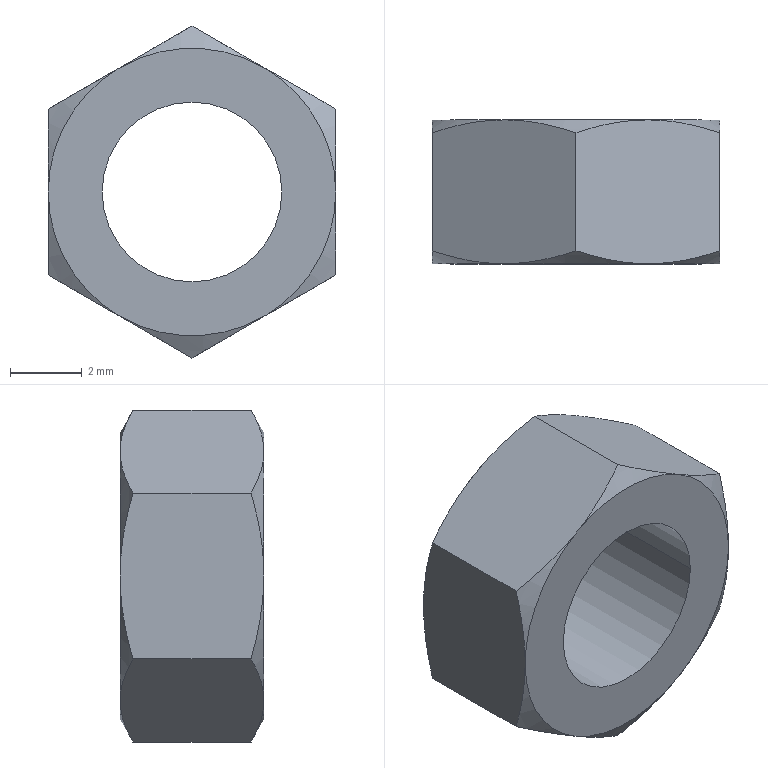Component | SolidWorks | PB_16x75_S_U_FA_M_2_0-1_164nut1-1 | 1 solid | 22 faces | box 8 x 4 x 9.24 mm | volume 142 mm3 | cone 12 | plane 8 | cylinder 2 | commonest cylinder face diameters 5 x2
build123d program:
from build123d import *

# Parameters (mm, degrees)
EXTRUDE1_DEPTH          = 2
EXTRUDE1_DEPTH_BACK     = 2
SKETCH3_W               = 16
SKETCH3_H               = 16
CUT_EXTRUDE1_DEPTH      = 7.429
CUT_EXTRUDE1_DEPTH_BACK = 7.429
SKETCH4_R               = 2.5


with BuildPart() as part:
    # Sketch1 → Revolve1 (revolve)
    with BuildSketch(Plane.XY, mode=Mode.PRIVATE) as revolve1_sk:
        Polygon((-2, 0), (-2, 4), (-1.538, 4.8), (1.538, 4.8), (2, 4), (2, 0), align=None)
    revolve(revolve1_sk.sketch.rotate(Axis((2, 0, 0), (-1, 0, 0)), 270), axis=Axis((2, 0, 0), (-1, 0, 0)))

    # Sketch2 → Cut-Revolve1 (revolve, cut)
    with BuildSketch(Plane.XY, mode=Mode.PRIVATE) as cut_revolve1_sk:
        Polygon((-2, 0), (-2, 2.5), (-1.567, 2.067), (1.567, 2.067), (2, 2.5), (2, 0), align=None)
    revolve(cut_revolve1_sk.sketch.rotate(Axis((2, 0, 0), (-1, 0, 0)), 270), axis=Axis((2, 0, 0), (-1, 0, 0)), mode=Mode.SUBTRACT)

    # Sketch3 → Extrude1 (cut, two sides: drawn at the far end of the back side and taken through both)
    with BuildSketch(Plane(origin=(0, 0, 0), x_dir=(0, 0, -1), z_dir=(1, 0, 0)).offset(-EXTRUDE1_DEPTH_BACK)):
        Rectangle(SKETCH3_W, SKETCH3_H)
        Polygon((-4, 2.309), (-4, -2.309), (0, -4.619), (4, -2.309), (4, 2.309), (0, 4.619), align=None, mode=Mode.SUBTRACT)
    extrude(amount=EXTRUDE1_DEPTH + EXTRUDE1_DEPTH_BACK, mode=Mode.SUBTRACT)

    # Sketch4 → Cut-Extrude1 (cut, two sides: drawn at the far end of the back side and taken through both)
    with BuildSketch(Plane(origin=(0, 0, 0), x_dir=(0, 0, -1), z_dir=(1, 0, 0)).offset(-CUT_EXTRUDE1_DEPTH_BACK)):
        Circle(SKETCH4_R)
    extrude(amount=CUT_EXTRUDE1_DEPTH + CUT_EXTRUDE1_DEPTH_BACK, mode=Mode.SUBTRACT)


solid = part.part

# Placed as in the assembly
solid = solid.moved(Location((45, -241, 55), (90, -90, 0)))
STEP:
#1=COLOUR_RGB('',0.7922,0.8196,0.9333);
#2=FILL_AREA_STYLE_COLOUR('',#1);
#3=FILL_AREA_STYLE('',(#2));
#4=SURFACE_STYLE_FILL_AREA(#3);
#5=SURFACE_SIDE_STYLE('',(#4));
#6=SURFACE_STYLE_USAGE(.BOTH.,#5);
#7=PRESENTATION_STYLE_ASSIGNMENT((#6));
#8=CARTESIAN_POINT('',(1.673,-9.567,2.165));
#9=VERTEX_POINT('',#8);
#10=CARTESIAN_POINT('',(1.87,-9.567,2.165));
#11=VERTEX_POINT('',#10);
#12=CARTESIAN_POINT('',(1.772,-9.567,2.165));
#13=DIRECTION('',(0.,1.,0.));
#14=DIRECTION('',(1.,0.,0.));
#15=AXIS2_PLACEMENT_3D('',#12,#13,#14);
#16=CIRCLE('',#15,0.09843);
#17=EDGE_CURVE('',#9,#11,#16,.T.);
#18=ORIENTED_EDGE('',*,*,#17,.F.);
#19=CARTESIAN_POINT('',(1.673,-9.409,2.165));
#20=VERTEX_POINT('',#19);
#21=CARTESIAN_POINT('',(1.673,-9.567,2.165));
#22=DIRECTION('',(0.,1.,0.));
#23=VECTOR('',#22,39.37);
#24=LINE('',#21,#23);
#25=EDGE_CURVE('',#9,#20,#24,.T.);
#26=ORIENTED_EDGE('',*,*,#25,.T.);
#27=CARTESIAN_POINT('',(1.87,-9.409,2.165));
#28=VERTEX_POINT('',#27);
#29=CARTESIAN_POINT('',(1.772,-9.409,2.165));
#30=DIRECTION('',(0.,1.,0.));
#31=DIRECTION('',(1.,0.,0.));
#32=AXIS2_PLACEMENT_3D('',#29,#30,#31);
#33=CIRCLE('',#32,0.09843);
#34=EDGE_CURVE('',#20,#28,#33,.T.);
#35=ORIENTED_EDGE('',*,*,#34,.T.);
#36=CARTESIAN_POINT('',(1.87,-9.567,2.165));
#37=DIRECTION('',(0.,1.,0.));
#38=VECTOR('',#37,39.37);
#39=LINE('',#36,#38);
#40=EDGE_CURVE('',#11,#28,#39,.T.);
#41=ORIENTED_EDGE('',*,*,#40,.F.);
#42=EDGE_LOOP('',(#18,#26,#35,#41));
#43=FACE_OUTER_BOUND('',#42,.T.);
#44=CARTESIAN_POINT('',(1.772,-9.567,2.165));
#45=DIRECTION('',(0.,1.,0.));
#46=DIRECTION('',(1.,0.,0.));
#47=AXIS2_PLACEMENT_3D('',#44,#45,#46);
#48=CYLINDRICAL_SURFACE('',#47,0.09843);
#49=ADVANCED_FACE('',(#43),#48,.F.);
#50=CARTESIAN_POINT('',(1.929,-9.553,2.256));
#51=VERTEX_POINT('',#50);
#52=CARTESIAN_POINT('',(1.929,-9.567,2.165));
#53=VERTEX_POINT('',#52);
#54=CARTESIAN_POINT('',(1.929,-9.553,2.256));
#55=CARTESIAN_POINT('',(1.929,-9.557,2.241));
#56=CARTESIAN_POINT('',(1.929,-9.561,2.226));
#57=CARTESIAN_POINT('',(1.929,-9.566,2.196));
#58=CARTESIAN_POINT('',(1.929,-9.567,2.181));
#59=CARTESIAN_POINT('',(1.929,-9.567,2.165));
#60=B_SPLINE_CURVE_WITH_KNOTS('',3,(#54,#55,#56,#57,#58,#59),.UNSPECIFIED.,.F.,.F.,(4,2,4),(0.004136,0.005305,0.006473),.UNSPECIFIED.);
#61=EDGE_CURVE('',#51,#53,#60,.T.);
#62=ORIENTED_EDGE('',*,*,#61,.F.);
#63=CARTESIAN_POINT('',(1.85,-9.567,2.302));
#64=VERTEX_POINT('',#63);
#65=CARTESIAN_POINT('',(1.85,-9.567,2.302));
#66=CARTESIAN_POINT('',(1.864,-9.567,2.294));
#67=CARTESIAN_POINT('',(1.877,-9.566,2.286));
#68=CARTESIAN_POINT('',(1.903,-9.561,2.271));
#69=CARTESIAN_POINT('',(1.916,-9.557,2.264));
#70=CARTESIAN_POINT('',(1.929,-9.553,2.256));
#71=B_SPLINE_CURVE_WITH_KNOTS('',3,(#65,#66,#67,#68,#69,#70),.UNSPECIFIED.,.F.,.F.,(4,2,4),(0.002337,0.003501,0.004665),.UNSPECIFIED.);
#72=EDGE_CURVE('',#64,#51,#71,.T.);
#73=ORIENTED_EDGE('',*,*,#72,.F.);
#74=CARTESIAN_POINT('',(1.772,-9.567,2.165));
#75=DIRECTION('',(0.,-1.,0.));
#76=DIRECTION('',(-1.,0.,0.));
#77=AXIS2_PLACEMENT_3D('',#74,#75,#76);
#78=CIRCLE('',#77,0.1575);
#79=EDGE_CURVE('',#53,#64,#78,.T.);
#80=ORIENTED_EDGE('',*,*,#79,.F.);
#81=EDGE_LOOP('',(#62,#73,#80));
#82=FACE_OUTER_BOUND('',#81,.T.);
#83=CARTESIAN_POINT('',(1.772,-9.549,2.165));
#84=DIRECTION('',(0.,1.,0.));
#85=DIRECTION('',(1.,0.,0.));
#86=AXIS2_PLACEMENT_3D('',#83,#84,#85);
#87=CONICAL_SURFACE('',#86,0.189,1.047);
#88=ADVANCED_FACE('',(#82),#87,.T.);
#89=CARTESIAN_POINT('',(1.929,-9.553,2.074));
#90=VERTEX_POINT('',#89);
#91=CARTESIAN_POINT('',(1.929,-9.567,2.165));
#92=CARTESIAN_POINT('',(1.929,-9.567,2.15));
#93=CARTESIAN_POINT('',(1.929,-9.566,2.134));
#94=CARTESIAN_POINT('',(1.929,-9.561,2.104));
#95=CARTESIAN_POINT('',(1.929,-9.557,2.089));
#96=CARTESIAN_POINT('',(1.929,-9.553,2.074));
#97=B_SPLINE_CURVE_WITH_KNOTS('',3,(#91,#92,#93,#94,#95,#96),.UNSPECIFIED.,.F.,.F.,(4,2,4),(0.006473,0.007642,0.008811),.UNSPECIFIED.);
#98=EDGE_CURVE('',#53,#90,#97,.T.);
#99=ORIENTED_EDGE('',*,*,#98,.F.);
#100=CARTESIAN_POINT('',(1.85,-9.567,2.029));
#101=VERTEX_POINT('',#100);
#102=CARTESIAN_POINT('',(1.772,-9.567,2.165));
#103=DIRECTION('',(0.,-1.,0.));
#104=DIRECTION('',(-1.,0.,0.));
#105=AXIS2_PLACEMENT_3D('',#102,#103,#104);
#106=CIRCLE('',#105,0.1575);
#107=EDGE_CURVE('',#101,#53,#106,.T.);
#108=ORIENTED_EDGE('',*,*,#107,.F.);
#109=CARTESIAN_POINT('',(1.929,-9.553,2.074));
#110=CARTESIAN_POINT('',(1.903,-9.561,2.06));
#111=CARTESIAN_POINT('',(1.877,-9.567,2.044));
#112=CARTESIAN_POINT('',(1.85,-9.567,2.029));
#113=B_SPLINE_CURVE_WITH_KNOTS('',3,(#109,#110,#111,#112),.UNSPECIFIED.,.F.,.F.,(4,4),(0.00000024,0.002337),.UNSPECIFIED.);
#114=EDGE_CURVE('',#90,#101,#113,.T.);
#115=ORIENTED_EDGE('',*,*,#114,.F.);
#116=EDGE_LOOP('',(#99,#108,#115));
#117=FACE_OUTER_BOUND('',#116,.T.);
#118=CARTESIAN_POINT('',(1.772,-9.549,2.165));
#119=DIRECTION('',(0.,1.,0.));
#120=DIRECTION('',(1.,0.,0.));
#121=AXIS2_PLACEMENT_3D('',#118,#119,#120);
#122=CONICAL_SURFACE('',#121,0.189,1.047);
#123=ADVANCED_FACE('',(#117),#122,.T.);
#124=CARTESIAN_POINT('',(1.772,-9.553,1.984));
#125=VERTEX_POINT('',#124);
#126=CARTESIAN_POINT('',(1.85,-9.567,2.029));
#127=CARTESIAN_POINT('',(1.837,-9.567,2.021));
#128=CARTESIAN_POINT('',(1.824,-9.566,2.014));
#129=CARTESIAN_POINT('',(1.797,-9.561,1.998));
#130=CARTESIAN_POINT('',(1.785,-9.557,1.991));
#131=CARTESIAN_POINT('',(1.772,-9.553,1.984));
#132=B_SPLINE_CURVE_WITH_KNOTS('',3,(#126,#127,#128,#129,#130,#131),.UNSPECIFIED.,.F.,.F.,(4,2,4),(0.002337,0.003501,0.004665),.UNSPECIFIED.);
#133=EDGE_CURVE('',#101,#125,#132,.T.);
#134=ORIENTED_EDGE('',*,*,#133,.F.);
#135=CARTESIAN_POINT('',(1.693,-9.567,2.029));
#136=VERTEX_POINT('',#135);
#137=CARTESIAN_POINT('',(1.772,-9.567,2.165));
#138=DIRECTION('',(0.,-1.,0.));
#139=DIRECTION('',(-1.,0.,0.));
#140=AXIS2_PLACEMENT_3D('',#137,#138,#139);
#141=CIRCLE('',#140,0.1575);
#142=EDGE_CURVE('',#136,#101,#141,.T.);
#143=ORIENTED_EDGE('',*,*,#142,.F.);
#144=CARTESIAN_POINT('',(1.772,-9.553,1.984));
#145=CARTESIAN_POINT('',(1.746,-9.561,1.998));
#146=CARTESIAN_POINT('',(1.72,-9.567,2.013));
#147=CARTESIAN_POINT('',(1.693,-9.567,2.029));
#148=B_SPLINE_CURVE_WITH_KNOTS('',3,(#144,#145,#146,#147),.UNSPECIFIED.,.F.,.F.,(4,4),(0.00000024,0.002337),.UNSPECIFIED.);
#149=EDGE_CURVE('',#125,#136,#148,.T.);
#150=ORIENTED_EDGE('',*,*,#149,.F.);
#151=EDGE_LOOP('',(#134,#143,#150));
#152=FACE_OUTER_BOUND('',#151,.T.);
#153=CARTESIAN_POINT('',(1.772,-9.549,2.165));
#154=DIRECTION('',(0.,1.,0.));
#155=DIRECTION('',(1.,0.,0.));
#156=AXIS2_PLACEMENT_3D('',#153,#154,#155);
#157=CONICAL_SURFACE('',#156,0.189,1.047);
#158=ADVANCED_FACE('',(#152),#157,.T.);
#159=CARTESIAN_POINT('',(1.772,-9.553,2.347));
#160=VERTEX_POINT('',#159);
#161=CARTESIAN_POINT('',(1.772,-9.553,2.347));
#162=CARTESIAN_POINT('',(1.797,-9.561,2.332));
#163=CARTESIAN_POINT('',(1.824,-9.567,2.317));
#164=CARTESIAN_POINT('',(1.85,-9.567,2.302));
#165=B_SPLINE_CURVE_WITH_KNOTS('',3,(#161,#162,#163,#164),.UNSPECIFIED.,.F.,.F.,(4,4),(0.00000024,0.002337),.UNSPECIFIED.);
#166=EDGE_CURVE('',#160,#64,#165,.T.);
#167=ORIENTED_EDGE('',*,*,#166,.F.);
#168=CARTESIAN_POINT('',(1.693,-9.567,2.302));
#169=VERTEX_POINT('',#168);
#170=CARTESIAN_POINT('',(1.693,-9.567,2.302));
#171=CARTESIAN_POINT('',(1.706,-9.567,2.309));
#172=CARTESIAN_POINT('',(1.72,-9.566,2.317));
#173=CARTESIAN_POINT('',(1.746,-9.561,2.332));
#174=CARTESIAN_POINT('',(1.759,-9.557,2.34));
#175=CARTESIAN_POINT('',(1.772,-9.553,2.347));
#176=B_SPLINE_CURVE_WITH_KNOTS('',3,(#170,#171,#172,#173,#174,#175),.UNSPECIFIED.,.F.,.F.,(4,2,4),(0.002337,0.003501,0.004665),.UNSPECIFIED.);
#177=EDGE_CURVE('',#169,#160,#176,.T.);
#178=ORIENTED_EDGE('',*,*,#177,.F.);
#179=CARTESIAN_POINT('',(1.772,-9.567,2.165));
#180=DIRECTION('',(0.,-1.,0.));
#181=DIRECTION('',(-1.,0.,0.));
#182=AXIS2_PLACEMENT_3D('',#179,#180,#181);
#183=CIRCLE('',#182,0.1575);
#184=EDGE_CURVE('',#64,#169,#183,.T.);
#185=ORIENTED_EDGE('',*,*,#184,.F.);
#186=EDGE_LOOP('',(#167,#178,#185));
#187=FACE_OUTER_BOUND('',#186,.T.);
#188=CARTESIAN_POINT('',(1.772,-9.549,2.165));
#189=DIRECTION('',(0.,1.,0.));
#190=DIRECTION('',(1.,0.,0.));
#191=AXIS2_PLACEMENT_3D('',#188,#189,#190);
#192=CONICAL_SURFACE('',#191,0.189,1.047);
#193=ADVANCED_FACE('',(#187),#192,.T.);
#194=CARTESIAN_POINT('',(1.614,-9.553,2.074));
#195=VERTEX_POINT('',#194);
#196=CARTESIAN_POINT('',(1.693,-9.567,2.029));
#197=CARTESIAN_POINT('',(1.68,-9.567,2.037));
#198=CARTESIAN_POINT('',(1.666,-9.566,2.044));
#199=CARTESIAN_POINT('',(1.64,-9.561,2.06));
#200=CARTESIAN_POINT('',(1.627,-9.557,2.067));
#201=CARTESIAN_POINT('',(1.614,-9.553,2.074));
#202=B_SPLINE_CURVE_WITH_KNOTS('',3,(#196,#197,#198,#199,#200,#201),.UNSPECIFIED.,.F.,.F.,(4,2,4),(0.002337,0.003501,0.004665),.UNSPECIFIED.);
#203=EDGE_CURVE('',#136,#195,#202,.T.);
#204=ORIENTED_EDGE('',*,*,#203,.F.);
#205=CARTESIAN_POINT('',(1.614,-9.567,2.165));
#206=VERTEX_POINT('',#205);
#207=CARTESIAN_POINT('',(1.772,-9.567,2.165));
#208=DIRECTION('',(0.,-1.,0.));
#209=DIRECTION('',(-1.,0.,0.));
#210=AXIS2_PLACEMENT_3D('',#207,#208,#209);
#211=CIRCLE('',#210,0.1575);
#212=EDGE_CURVE('',#206,#136,#211,.T.);
#213=ORIENTED_EDGE('',*,*,#212,.F.);
#214=CARTESIAN_POINT('',(1.614,-9.553,2.074));
#215=CARTESIAN_POINT('',(1.614,-9.557,2.089));
#216=CARTESIAN_POINT('',(1.614,-9.561,2.104));
#217=CARTESIAN_POINT('',(1.614,-9.566,2.134));
#218=CARTESIAN_POINT('',(1.614,-9.567,2.15));
#219=CARTESIAN_POINT('',(1.614,-9.567,2.165));
#220=B_SPLINE_CURVE_WITH_KNOTS('',3,(#214,#215,#216,#217,#218,#219),.UNSPECIFIED.,.F.,.F.,(4,2,4),(0.01014,0.01131,0.01248),.UNSPECIFIED.);
#221=EDGE_CURVE('',#195,#206,#220,.T.);
#222=ORIENTED_EDGE('',*,*,#221,.F.);
#223=EDGE_LOOP('',(#204,#213,#222));
#224=FACE_OUTER_BOUND('',#223,.T.);
#225=CARTESIAN_POINT('',(1.772,-9.549,2.165));
#226=DIRECTION('',(0.,1.,0.));
#227=DIRECTION('',(1.,0.,0.));
#228=AXIS2_PLACEMENT_3D('',#225,#226,#227);
#229=CONICAL_SURFACE('',#228,0.189,1.047);
#230=ADVANCED_FACE('',(#224),#229,.T.);
#231=CARTESIAN_POINT('',(1.614,-9.553,2.256));
#232=VERTEX_POINT('',#231);
#233=CARTESIAN_POINT('',(1.614,-9.553,2.256));
#234=CARTESIAN_POINT('',(1.64,-9.561,2.271));
#235=CARTESIAN_POINT('',(1.666,-9.567,2.286));
#236=CARTESIAN_POINT('',(1.693,-9.567,2.302));
#237=B_SPLINE_CURVE_WITH_KNOTS('',3,(#233,#234,#235,#236),.UNSPECIFIED.,.F.,.F.,(4,4),(0.00000024,0.002337),.UNSPECIFIED.);
#238=EDGE_CURVE('',#232,#169,#237,.T.);
#239=ORIENTED_EDGE('',*,*,#238,.F.);
#240=CARTESIAN_POINT('',(1.614,-9.567,2.165));
#241=CARTESIAN_POINT('',(1.614,-9.567,2.181));
#242=CARTESIAN_POINT('',(1.614,-9.566,2.196));
#243=CARTESIAN_POINT('',(1.614,-9.561,2.226));
#244=CARTESIAN_POINT('',(1.614,-9.557,2.241));
#245=CARTESIAN_POINT('',(1.614,-9.553,2.256));
#246=B_SPLINE_CURVE_WITH_KNOTS('',3,(#240,#241,#242,#243,#244,#245),.UNSPECIFIED.,.F.,.F.,(4,2,4),(0.01248,0.01365,0.01482),.UNSPECIFIED.);
#247=EDGE_CURVE('',#206,#232,#246,.T.);
#248=ORIENTED_EDGE('',*,*,#247,.F.);
#249=CARTESIAN_POINT('',(1.772,-9.567,2.165));
#250=DIRECTION('',(0.,-1.,0.));
#251=DIRECTION('',(-1.,0.,0.));
#252=AXIS2_PLACEMENT_3D('',#249,#250,#251);
#253=CIRCLE('',#252,0.1575);
#254=EDGE_CURVE('',#169,#206,#253,.T.);
#255=ORIENTED_EDGE('',*,*,#254,.F.);
#256=EDGE_LOOP('',(#239,#248,#255));
#257=FACE_OUTER_BOUND('',#256,.T.);
#258=CARTESIAN_POINT('',(1.772,-9.549,2.165));
#259=DIRECTION('',(0.,1.,0.));
#260=DIRECTION('',(1.,0.,0.));
#261=AXIS2_PLACEMENT_3D('',#258,#259,#260);
#262=CONICAL_SURFACE('',#261,0.189,1.047);
#263=ADVANCED_FACE('',(#257),#262,.T.);
#264=CARTESIAN_POINT('',(1.614,-9.424,2.074));
#265=VERTEX_POINT('',#264);
#266=CARTESIAN_POINT('',(1.693,-9.409,2.029));
#267=VERTEX_POINT('',#266);
#268=CARTESIAN_POINT('',(1.614,-9.424,2.074));
#269=CARTESIAN_POINT('',(1.64,-9.415,2.06));
#270=CARTESIAN_POINT('',(1.666,-9.409,2.044));
#271=CARTESIAN_POINT('',(1.693,-9.409,2.029));
#272=B_SPLINE_CURVE_WITH_KNOTS('',3,(#268,#269,#270,#271),.UNSPECIFIED.,.F.,.F.,(4,4),(0.00000024,0.002337),.UNSPECIFIED.);
#273=EDGE_CURVE('',#265,#267,#272,.T.);
#274=ORIENTED_EDGE('',*,*,#273,.F.);
#275=CARTESIAN_POINT('',(1.614,-9.409,2.165));
#276=VERTEX_POINT('',#275);
#277=CARTESIAN_POINT('',(1.614,-9.409,2.165));
#278=CARTESIAN_POINT('',(1.614,-9.409,2.15));
#279=CARTESIAN_POINT('',(1.614,-9.411,2.134));
#280=CARTESIAN_POINT('',(1.614,-9.416,2.104));
#281=CARTESIAN_POINT('',(1.614,-9.419,2.089));
#282=CARTESIAN_POINT('',(1.614,-9.424,2.074));
#283=B_SPLINE_CURVE_WITH_KNOTS('',3,(#277,#278,#279,#280,#281,#282),.UNSPECIFIED.,.F.,.F.,(4,2,4),(0.006473,0.007642,0.008811),.UNSPECIFIED.);
#284=EDGE_CURVE('',#276,#265,#283,.T.);
#285=ORIENTED_EDGE('',*,*,#284,.F.);
#286=CARTESIAN_POINT('',(1.772,-9.409,2.165));
#287=DIRECTION('',(0.,-1.,0.));
#288=DIRECTION('',(-1.,0.,0.));
#289=AXIS2_PLACEMENT_3D('',#286,#287,#288);
#290=CIRCLE('',#289,0.1575);
#291=EDGE_CURVE('',#276,#267,#290,.T.);
#292=ORIENTED_EDGE('',*,*,#291,.T.);
#293=EDGE_LOOP('',(#274,#285,#292));
#294=FACE_OUTER_BOUND('',#293,.T.);
#295=CARTESIAN_POINT('',(1.772,-9.409,2.165));
#296=DIRECTION('',(0.,-1.,0.));
#297=DIRECTION('',(-1.,0.,0.));
#298=AXIS2_PLACEMENT_3D('',#295,#296,#297);
#299=CONICAL_SURFACE('',#298,0.1575,1.047);
#300=ADVANCED_FACE('',(#294),#299,.T.);
#301=CARTESIAN_POINT('',(1.772,-9.424,1.984));
#302=VERTEX_POINT('',#301);
#303=CARTESIAN_POINT('',(1.693,-9.409,2.029));
#304=CARTESIAN_POINT('',(1.706,-9.409,2.021));
#305=CARTESIAN_POINT('',(1.72,-9.411,2.014));
#306=CARTESIAN_POINT('',(1.746,-9.416,1.998));
#307=CARTESIAN_POINT('',(1.759,-9.419,1.991));
#308=CARTESIAN_POINT('',(1.772,-9.424,1.984));
#309=B_SPLINE_CURVE_WITH_KNOTS('',3,(#303,#304,#305,#306,#307,#308),.UNSPECIFIED.,.F.,.F.,(4,2,4),(0.002337,0.003501,0.004665),.UNSPECIFIED.);
#310=EDGE_CURVE('',#267,#302,#309,.T.);
#311=ORIENTED_EDGE('',*,*,#310,.F.);
#312=CARTESIAN_POINT('',(1.85,-9.409,2.029));
#313=VERTEX_POINT('',#312);
#314=CARTESIAN_POINT('',(1.772,-9.409,2.165));
#315=DIRECTION('',(0.,-1.,0.));
#316=DIRECTION('',(-1.,0.,0.));
#317=AXIS2_PLACEMENT_3D('',#314,#315,#316);
#318=CIRCLE('',#317,0.1575);
#319=EDGE_CURVE('',#267,#313,#318,.T.);
#320=ORIENTED_EDGE('',*,*,#319,.T.);
#321=CARTESIAN_POINT('',(1.772,-9.424,1.984));
#322=CARTESIAN_POINT('',(1.797,-9.415,1.998));
#323=CARTESIAN_POINT('',(1.824,-9.409,2.013));
#324=CARTESIAN_POINT('',(1.85,-9.409,2.029));
#325=B_SPLINE_CURVE_WITH_KNOTS('',3,(#321,#322,#323,#324),.UNSPECIFIED.,.F.,.F.,(4,4),(0.00000024,0.002337),.UNSPECIFIED.);
#326=EDGE_CURVE('',#302,#313,#325,.T.);
#327=ORIENTED_EDGE('',*,*,#326,.F.);
#328=EDGE_LOOP('',(#311,#320,#327));
#329=FACE_OUTER_BOUND('',#328,.T.);
#330=CARTESIAN_POINT('',(1.772,-9.409,2.165));
#331=DIRECTION('',(0.,-1.,0.));
#332=DIRECTION('',(-1.,0.,0.));
#333=AXIS2_PLACEMENT_3D('',#330,#331,#332);
#334=CONICAL_SURFACE('',#333,0.1575,1.047);
#335=ADVANCED_FACE('',(#329),#334,.T.);
#336=CARTESIAN_POINT('',(1.929,-9.424,2.074));
#337=VERTEX_POINT('',#336);
#338=CARTESIAN_POINT('',(1.85,-9.409,2.029));
#339=CARTESIAN_POINT('',(1.864,-9.409,2.037));
#340=CARTESIAN_POINT('',(1.877,-9.411,2.044));
#341=CARTESIAN_POINT('',(1.903,-9.416,2.06));
#342=CARTESIAN_POINT('',(1.916,-9.419,2.067));
#343=CARTESIAN_POINT('',(1.929,-9.424,2.074));
#344=B_SPLINE_CURVE_WITH_KNOTS('',3,(#338,#339,#340,#341,#342,#343),.UNSPECIFIED.,.F.,.F.,(4,2,4),(0.002337,0.003501,0.004665),.UNSPECIFIED.);
#345=EDGE_CURVE('',#313,#337,#344,.T.);
#346=ORIENTED_EDGE('',*,*,#345,.F.);
#347=CARTESIAN_POINT('',(1.929,-9.409,2.165));
#348=VERTEX_POINT('',#347);
#349=CARTESIAN_POINT('',(1.772,-9.409,2.165));
#350=DIRECTION('',(0.,-1.,0.));
#351=DIRECTION('',(-1.,0.,0.));
#352=AXIS2_PLACEMENT_3D('',#349,#350,#351);
#353=CIRCLE('',#352,0.1575);
#354=EDGE_CURVE('',#313,#348,#353,.T.);
#355=ORIENTED_EDGE('',*,*,#354,.T.);
#356=CARTESIAN_POINT('',(1.929,-9.424,2.074));
#357=CARTESIAN_POINT('',(1.929,-9.419,2.089));
#358=CARTESIAN_POINT('',(1.929,-9.416,2.104));
#359=CARTESIAN_POINT('',(1.929,-9.411,2.134));
#360=CARTESIAN_POINT('',(1.929,-9.409,2.15));
#361=CARTESIAN_POINT('',(1.929,-9.409,2.165));
#362=B_SPLINE_CURVE_WITH_KNOTS('',3,(#356,#357,#358,#359,#360,#361),.UNSPECIFIED.,.F.,.F.,(4,2,4),(0.01014,0.01131,0.01248),.UNSPECIFIED.);
#363=EDGE_CURVE('',#337,#348,#362,.T.);
#364=ORIENTED_EDGE('',*,*,#363,.F.);
#365=EDGE_LOOP('',(#346,#355,#364));
#366=FACE_OUTER_BOUND('',#365,.T.);
#367=CARTESIAN_POINT('',(1.772,-9.409,2.165));
#368=DIRECTION('',(0.,-1.,0.));
#369=DIRECTION('',(-1.,0.,0.));
#370=AXIS2_PLACEMENT_3D('',#367,#368,#369);
#371=CONICAL_SURFACE('',#370,0.1575,1.047);
#372=ADVANCED_FACE('',(#366),#371,.T.);
#373=CARTESIAN_POINT('',(1.929,-9.424,2.256));
#374=VERTEX_POINT('',#373);
#375=CARTESIAN_POINT('',(1.929,-9.409,2.165));
#376=CARTESIAN_POINT('',(1.929,-9.409,2.181));
#377=CARTESIAN_POINT('',(1.929,-9.411,2.196));
#378=CARTESIAN_POINT('',(1.929,-9.416,2.226));
#379=CARTESIAN_POINT('',(1.929,-9.419,2.241));
#380=CARTESIAN_POINT('',(1.929,-9.424,2.256));
#381=B_SPLINE_CURVE_WITH_KNOTS('',3,(#375,#376,#377,#378,#379,#380),.UNSPECIFIED.,.F.,.F.,(4,2,4),(0.01248,0.01365,0.01482),.UNSPECIFIED.);
#382=EDGE_CURVE('',#348,#374,#381,.T.);
#383=ORIENTED_EDGE('',*,*,#382,.F.);
#384=CARTESIAN_POINT('',(1.85,-9.409,2.302));
#385=VERTEX_POINT('',#384);
#386=CARTESIAN_POINT('',(1.772,-9.409,2.165));
#387=DIRECTION('',(0.,-1.,0.));
#388=DIRECTION('',(-1.,0.,0.));
#389=AXIS2_PLACEMENT_3D('',#386,#387,#388);
#390=CIRCLE('',#389,0.1575);
#391=EDGE_CURVE('',#348,#385,#390,.T.);
#392=ORIENTED_EDGE('',*,*,#391,.T.);
#393=CARTESIAN_POINT('',(1.929,-9.424,2.256));
#394=CARTESIAN_POINT('',(1.903,-9.415,2.271));
#395=CARTESIAN_POINT('',(1.877,-9.409,2.286));
#396=CARTESIAN_POINT('',(1.85,-9.409,2.302));
#397=B_SPLINE_CURVE_WITH_KNOTS('',3,(#393,#394,#395,#396),.UNSPECIFIED.,.F.,.F.,(4,4),(0.00000024,0.002337),.UNSPECIFIED.);
#398=EDGE_CURVE('',#374,#385,#397,.T.);
#399=ORIENTED_EDGE('',*,*,#398,.F.);
#400=EDGE_LOOP('',(#383,#392,#399));
#401=FACE_OUTER_BOUND('',#400,.T.);
#402=CARTESIAN_POINT('',(1.772,-9.409,2.165));
#403=DIRECTION('',(0.,-1.,0.));
#404=DIRECTION('',(-1.,0.,0.));
#405=AXIS2_PLACEMENT_3D('',#402,#403,#404);
#406=CONICAL_SURFACE('',#405,0.1575,1.047);
#407=ADVANCED_FACE('',(#401),#406,.T.);
#408=CARTESIAN_POINT('',(1.772,-9.424,2.347));
#409=VERTEX_POINT('',#408);
#410=CARTESIAN_POINT('',(1.85,-9.409,2.302));
#411=CARTESIAN_POINT('',(1.837,-9.409,2.309));
#412=CARTESIAN_POINT('',(1.824,-9.411,2.317));
#413=CARTESIAN_POINT('',(1.797,-9.416,2.332));
#414=CARTESIAN_POINT('',(1.785,-9.419,2.34));
#415=CARTESIAN_POINT('',(1.772,-9.424,2.347));
#416=B_SPLINE_CURVE_WITH_KNOTS('',3,(#410,#411,#412,#413,#414,#415),.UNSPECIFIED.,.F.,.F.,(4,2,4),(0.002337,0.003501,0.004665),.UNSPECIFIED.);
#417=EDGE_CURVE('',#385,#409,#416,.T.);
#418=ORIENTED_EDGE('',*,*,#417,.F.);
#419=CARTESIAN_POINT('',(1.693,-9.409,2.302));
#420=VERTEX_POINT('',#419);
#421=CARTESIAN_POINT('',(1.772,-9.409,2.165));
#422=DIRECTION('',(0.,-1.,0.));
#423=DIRECTION('',(-1.,0.,0.));
#424=AXIS2_PLACEMENT_3D('',#421,#422,#423);
#425=CIRCLE('',#424,0.1575);
#426=EDGE_CURVE('',#385,#420,#425,.T.);
#427=ORIENTED_EDGE('',*,*,#426,.T.);
#428=CARTESIAN_POINT('',(1.772,-9.424,2.347));
#429=CARTESIAN_POINT('',(1.746,-9.415,2.332));
#430=CARTESIAN_POINT('',(1.72,-9.409,2.317));
#431=CARTESIAN_POINT('',(1.693,-9.409,2.302));
#432=B_SPLINE_CURVE_WITH_KNOTS('',3,(#428,#429,#430,#431),.UNSPECIFIED.,.F.,.F.,(4,4),(0.00000024,0.002337),.UNSPECIFIED.);
#433=EDGE_CURVE('',#409,#420,#432,.T.);
#434=ORIENTED_EDGE('',*,*,#433,.F.);
#435=EDGE_LOOP('',(#418,#427,#434));
#436=FACE_OUTER_BOUND('',#435,.T.);
#437=CARTESIAN_POINT('',(1.772,-9.409,2.165));
#438=DIRECTION('',(0.,-1.,0.));
#439=DIRECTION('',(-1.,0.,0.));
#440=AXIS2_PLACEMENT_3D('',#437,#438,#439);
#441=CONICAL_SURFACE('',#440,0.1575,1.047);
#442=ADVANCED_FACE('',(#436),#441,.T.);
#443=CARTESIAN_POINT('',(1.614,-9.424,2.256));
#444=VERTEX_POINT('',#443);
#445=CARTESIAN_POINT('',(1.693,-9.409,2.302));
#446=CARTESIAN_POINT('',(1.68,-9.409,2.294));
#447=CARTESIAN_POINT('',(1.666,-9.411,2.286));
#448=CARTESIAN_POINT('',(1.64,-9.416,2.271));
#449=CARTESIAN_POINT('',(1.627,-9.419,2.264));
#450=CARTESIAN_POINT('',(1.614,-9.424,2.256));
#451=B_SPLINE_CURVE_WITH_KNOTS('',3,(#445,#446,#447,#448,#449,#450),.UNSPECIFIED.,.F.,.F.,(4,2,4),(0.002337,0.003501,0.004665),.UNSPECIFIED.);
#452=EDGE_CURVE('',#420,#444,#451,.T.);
#453=ORIENTED_EDGE('',*,*,#452,.F.);
#454=CARTESIAN_POINT('',(1.772,-9.409,2.165));
#455=DIRECTION('',(0.,-1.,0.));
#456=DIRECTION('',(-1.,0.,0.));
#457=AXIS2_PLACEMENT_3D('',#454,#455,#456);
#458=CIRCLE('',#457,0.1575);
#459=EDGE_CURVE('',#420,#276,#458,.T.);
#460=ORIENTED_EDGE('',*,*,#459,.T.);
#461=CARTESIAN_POINT('',(1.614,-9.424,2.256));
#462=CARTESIAN_POINT('',(1.614,-9.419,2.241));
#463=CARTESIAN_POINT('',(1.614,-9.416,2.226));
#464=CARTESIAN_POINT('',(1.614,-9.411,2.196));
#465=CARTESIAN_POINT('',(1.614,-9.409,2.181));
#466=CARTESIAN_POINT('',(1.614,-9.409,2.165));
#467=B_SPLINE_CURVE_WITH_KNOTS('',3,(#461,#462,#463,#464,#465,#466),.UNSPECIFIED.,.F.,.F.,(4,2,4),(0.004136,0.005305,0.006473),.UNSPECIFIED.);
#468=EDGE_CURVE('',#444,#276,#467,.T.);
#469=ORIENTED_EDGE('',*,*,#468,.F.);
#470=EDGE_LOOP('',(#453,#460,#469));
#471=FACE_OUTER_BOUND('',#470,.T.);
#472=CARTESIAN_POINT('',(1.772,-9.409,2.165));
#473=DIRECTION('',(0.,-1.,0.));
#474=DIRECTION('',(-1.,0.,0.));
#475=AXIS2_PLACEMENT_3D('',#472,#473,#474);
#476=CONICAL_SURFACE('',#475,0.1575,1.047);
#477=ADVANCED_FACE('',(#471),#476,.T.);
#478=ORIENTED_EDGE('',*,*,#212,.T.);
#479=ORIENTED_EDGE('',*,*,#142,.T.);
#480=ORIENTED_EDGE('',*,*,#107,.T.);
#481=ORIENTED_EDGE('',*,*,#79,.T.);
#482=ORIENTED_EDGE('',*,*,#184,.T.);
#483=ORIENTED_EDGE('',*,*,#254,.T.);
#484=EDGE_LOOP('',(#478,#479,#480,#481,#482,#483));
#485=FACE_OUTER_BOUND('',#484,.T.);
#486=CARTESIAN_POINT('',(1.772,-9.567,2.165));
#487=DIRECTION('',(0.,1.,0.));
#488=DIRECTION('',(1.,0.,0.));
#489=AXIS2_PLACEMENT_3D('',#486,#487,#488);
#490=CIRCLE('',#489,0.09843);
#491=EDGE_CURVE('',#11,#9,#490,.T.);
#492=ORIENTED_EDGE('',*,*,#491,.T.);
#493=ORIENTED_EDGE('',*,*,#17,.T.);
#494=EDGE_LOOP('',(#492,#493));
#495=FACE_BOUND('',#494,.T.);
#496=CARTESIAN_POINT('',(1.772,-9.567,2.165));
#497=DIRECTION('',(0.,1.,0.));
#498=DIRECTION('',(1.,0.,0.));
#499=AXIS2_PLACEMENT_3D('',#496,#497,#498);
#500=PLANE('',#499);
#501=ADVANCED_FACE('',(#485,#495),#500,.F.);
#502=ORIENTED_EDGE('',*,*,#291,.F.);
#503=ORIENTED_EDGE('',*,*,#459,.F.);
#504=ORIENTED_EDGE('',*,*,#426,.F.);
#505=ORIENTED_EDGE('',*,*,#391,.F.);
#506=ORIENTED_EDGE('',*,*,#354,.F.);
#507=ORIENTED_EDGE('',*,*,#319,.F.);
#508=EDGE_LOOP('',(#502,#503,#504,#505,#506,#507));
#509=FACE_OUTER_BOUND('',#508,.T.);
#510=CARTESIAN_POINT('',(1.772,-9.409,2.165));
#511=DIRECTION('',(0.,1.,0.));
#512=DIRECTION('',(1.,0.,0.));
#513=AXIS2_PLACEMENT_3D('',#510,#511,#512);
#514=CIRCLE('',#513,0.09843);
#515=EDGE_CURVE('',#28,#20,#514,.T.);
#516=ORIENTED_EDGE('',*,*,#515,.F.);
#517=ORIENTED_EDGE('',*,*,#34,.F.);
#518=EDGE_LOOP('',(#516,#517));
#519=FACE_BOUND('',#518,.T.);
#520=CARTESIAN_POINT('',(1.772,-9.409,2.008));
#521=DIRECTION('',(0.,-1.,0.));
#522=DIRECTION('',(-1.,0.,0.));
#523=AXIS2_PLACEMENT_3D('',#520,#521,#522);
#524=PLANE('',#523);
#525=ADVANCED_FACE('',(#509,#519),#524,.F.);
#526=ORIENTED_EDGE('',*,*,#149,.T.);
#527=ORIENTED_EDGE('',*,*,#203,.T.);
#528=CARTESIAN_POINT('',(1.614,-9.567,2.074));
#529=DIRECTION('',(0.,1.,0.));
#530=VECTOR('',#529,39.37);
#531=LINE('',#528,#530);
#532=EDGE_CURVE('',#195,#265,#531,.T.);
#533=ORIENTED_EDGE('',*,*,#532,.T.);
#534=ORIENTED_EDGE('',*,*,#273,.T.);
#535=ORIENTED_EDGE('',*,*,#310,.T.);
#536=CARTESIAN_POINT('',(1.772,-9.567,1.984));
#537=DIRECTION('',(0.,1.,0.));
#538=VECTOR('',#537,39.37);
#539=LINE('',#536,#538);
#540=EDGE_CURVE('',#125,#302,#539,.T.);
#541=ORIENTED_EDGE('',*,*,#540,.F.);
#542=EDGE_LOOP('',(#526,#527,#533,#534,#535,#541));
#543=FACE_OUTER_BOUND('',#542,.T.);
#544=CARTESIAN_POINT('',(1.772,-9.567,1.984));
#545=DIRECTION('',(-0.5,0.,-0.866));
#546=DIRECTION('',(-0.866,0.,0.5));
#547=AXIS2_PLACEMENT_3D('',#544,#545,#546);
#548=PLANE('',#547);
#549=ADVANCED_FACE('',(#543),#548,.T.);
#550=ORIENTED_EDGE('',*,*,#114,.T.);
#551=ORIENTED_EDGE('',*,*,#133,.T.);
#552=ORIENTED_EDGE('',*,*,#540,.T.);
#553=ORIENTED_EDGE('',*,*,#326,.T.);
#554=ORIENTED_EDGE('',*,*,#345,.T.);
#555=CARTESIAN_POINT('',(1.929,-9.567,2.074));
#556=DIRECTION('',(0.,1.,0.));
#557=VECTOR('',#556,39.37);
#558=LINE('',#555,#557);
#559=EDGE_CURVE('',#90,#337,#558,.T.);
#560=ORIENTED_EDGE('',*,*,#559,.F.);
#561=EDGE_LOOP('',(#550,#551,#552,#553,#554,#560));
#562=FACE_OUTER_BOUND('',#561,.T.);
#563=CARTESIAN_POINT('',(1.929,-9.567,2.074));
#564=DIRECTION('',(0.5,0.,-0.866));
#565=DIRECTION('',(-0.866,0.,-0.5));
#566=AXIS2_PLACEMENT_3D('',#563,#564,#565);
#567=PLANE('',#566);
#568=ADVANCED_FACE('',(#562),#567,.T.);
#569=ORIENTED_EDGE('',*,*,#61,.T.);
#570=ORIENTED_EDGE('',*,*,#98,.T.);
#571=ORIENTED_EDGE('',*,*,#559,.T.);
#572=ORIENTED_EDGE('',*,*,#363,.T.);
#573=ORIENTED_EDGE('',*,*,#382,.T.);
#574=CARTESIAN_POINT('',(1.929,-9.567,2.256));
#575=DIRECTION('',(0.,1.,0.));
#576=VECTOR('',#575,39.37);
#577=LINE('',#574,#576);
#578=EDGE_CURVE('',#51,#374,#577,.T.);
#579=ORIENTED_EDGE('',*,*,#578,.F.);
#580=EDGE_LOOP('',(#569,#570,#571,#572,#573,#579));
#581=FACE_OUTER_BOUND('',#580,.T.);
#582=CARTESIAN_POINT('',(1.929,-9.567,2.256));
#583=DIRECTION('',(1.,0.,0.));
#584=DIRECTION('',(0.,-1.,0.));
#585=AXIS2_PLACEMENT_3D('',#582,#583,#584);
#586=PLANE('',#585);
#587=ADVANCED_FACE('',(#581),#586,.T.);
#588=ORIENTED_EDGE('',*,*,#166,.T.);
#589=ORIENTED_EDGE('',*,*,#72,.T.);
#590=ORIENTED_EDGE('',*,*,#578,.T.);
#591=ORIENTED_EDGE('',*,*,#398,.T.);
#592=ORIENTED_EDGE('',*,*,#417,.T.);
#593=CARTESIAN_POINT('',(1.772,-9.567,2.347));
#594=DIRECTION('',(0.,1.,0.));
#595=VECTOR('',#594,39.37);
#596=LINE('',#593,#595);
#597=EDGE_CURVE('',#160,#409,#596,.T.);
#598=ORIENTED_EDGE('',*,*,#597,.F.);
#599=EDGE_LOOP('',(#588,#589,#590,#591,#592,#598));
#600=FACE_OUTER_BOUND('',#599,.T.);
#601=CARTESIAN_POINT('',(1.772,-9.567,2.347));
#602=DIRECTION('',(0.5,0.,0.866));
#603=DIRECTION('',(0.866,0.,-0.5));
#604=AXIS2_PLACEMENT_3D('',#601,#602,#603);
#605=PLANE('',#604);
#606=ADVANCED_FACE('',(#600),#605,.T.);
#607=ORIENTED_EDGE('',*,*,#238,.T.);
#608=ORIENTED_EDGE('',*,*,#177,.T.);
#609=ORIENTED_EDGE('',*,*,#597,.T.);
#610=ORIENTED_EDGE('',*,*,#433,.T.);
#611=ORIENTED_EDGE('',*,*,#452,.T.);
#612=CARTESIAN_POINT('',(1.614,-9.567,2.256));
#613=DIRECTION('',(0.,1.,0.));
#614=VECTOR('',#613,39.37);
#615=LINE('',#612,#614);
#616=EDGE_CURVE('',#232,#444,#615,.T.);
#617=ORIENTED_EDGE('',*,*,#616,.F.);
#618=EDGE_LOOP('',(#607,#608,#609,#610,#611,#617));
#619=FACE_OUTER_BOUND('',#618,.T.);
#620=CARTESIAN_POINT('',(1.614,-9.567,2.256));
#621=DIRECTION('',(-0.5,0.,0.866));
#622=DIRECTION('',(0.866,0.,0.5));
#623=AXIS2_PLACEMENT_3D('',#620,#621,#622);
#624=PLANE('',#623);
#625=ADVANCED_FACE('',(#619),#624,.T.);
#626=ORIENTED_EDGE('',*,*,#221,.T.);
#627=ORIENTED_EDGE('',*,*,#247,.T.);
#628=ORIENTED_EDGE('',*,*,#616,.T.);
#629=ORIENTED_EDGE('',*,*,#468,.T.);
#630=ORIENTED_EDGE('',*,*,#284,.T.);
#631=ORIENTED_EDGE('',*,*,#532,.F.);
#632=EDGE_LOOP('',(#626,#627,#628,#629,#630,#631));
#633=FACE_OUTER_BOUND('',#632,.T.);
#634=CARTESIAN_POINT('',(1.614,-9.567,2.074));
#635=DIRECTION('',(-1.,0.,0.));
#636=DIRECTION('',(0.,1.,0.));
#637=AXIS2_PLACEMENT_3D('',#634,#635,#636);
#638=PLANE('',#637);
#639=ADVANCED_FACE('',(#633),#638,.T.);
#640=ORIENTED_EDGE('',*,*,#25,.F.);
#641=ORIENTED_EDGE('',*,*,#491,.F.);
#642=ORIENTED_EDGE('',*,*,#40,.T.);
#643=ORIENTED_EDGE('',*,*,#515,.T.);
#644=EDGE_LOOP('',(#640,#641,#642,#643));
#645=FACE_OUTER_BOUND('',#644,.T.);
#646=CARTESIAN_POINT('',(1.772,-9.567,2.165));
#647=DIRECTION('',(0.,1.,0.));
#648=DIRECTION('',(1.,0.,0.));
#649=AXIS2_PLACEMENT_3D('',#646,#647,#648);
#650=CYLINDRICAL_SURFACE('',#649,0.09843);
#651=ADVANCED_FACE('',(#645),#650,.F.);
#652=CLOSED_SHELL('',(#49,#88,#123,#158,#193,#230,#263,#300,#335,#372,#407,#442,#477,#501,#525,#549,#568,#587,#606,#625,#639,#651));
#653=MANIFOLD_SOLID_BREP('',#652);
#654=STYLED_ITEM('',(#7),#653);
#655=PRESENTATION_LAYER_ASSIGNMENT('','',(#654));
#656=(LENGTH_UNIT()NAMED_UNIT(*)SI_UNIT($,.METRE.));
#657=LENGTH_MEASURE_WITH_UNIT(LENGTH_MEASURE(0.0254),#656);
#658=DIMENSIONAL_EXPONENTS(1.,0.,0.,0.,0.,0.,0.);
#659=(CONVERSION_BASED_UNIT('',#657)LENGTH_UNIT()NAMED_UNIT(#658));
#660=UNCERTAINTY_MEASURE_WITH_UNIT(LENGTH_MEASURE(0.00001),#659,'','');
#661=(NAMED_UNIT(*)PLANE_ANGLE_UNIT()SI_UNIT($,.RADIAN.));
#662=(NAMED_UNIT(*)SI_UNIT($,.STERADIAN.)SOLID_ANGLE_UNIT());
#663=(GEOMETRIC_REPRESENTATION_CONTEXT(3)GLOBAL_UNCERTAINTY_ASSIGNED_CONTEXT((#660))GLOBAL_UNIT_ASSIGNED_CONTEXT((#659,#661,#662))REPRESENTATION_CONTEXT('',''));
#664=MECHANICAL_DESIGN_GEOMETRIC_PRESENTATION_REPRESENTATION('',(#654),#663);
#665=CARTESIAN_POINT('',(0.,0.,0.));
#666=DIRECTION('',(0.,0.,1.));
#667=DIRECTION('',(1.,0.,0.));
#668=AXIS2_PLACEMENT_3D('',#665,#666,#667);
#669=(LENGTH_UNIT()NAMED_UNIT(*)SI_UNIT($,.METRE.));
#670=LENGTH_MEASURE_WITH_UNIT(LENGTH_MEASURE(0.0254),#669);
#671=DIMENSIONAL_EXPONENTS(1.,0.,0.,0.,0.,0.,0.);
#672=(CONVERSION_BASED_UNIT('',#670)LENGTH_UNIT()NAMED_UNIT(#671));
#673=UNCERTAINTY_MEASURE_WITH_UNIT(LENGTH_MEASURE(0.00001),#672,'','');
#674=(NAMED_UNIT(*)PLANE_ANGLE_UNIT()SI_UNIT($,.RADIAN.));
#675=(NAMED_UNIT(*)SI_UNIT($,.STERADIAN.)SOLID_ANGLE_UNIT());
#676=(GEOMETRIC_REPRESENTATION_CONTEXT(3)GLOBAL_UNCERTAINTY_ASSIGNED_CONTEXT((#673))GLOBAL_UNIT_ASSIGNED_CONTEXT((#672,#674,#675))REPRESENTATION_CONTEXT('',''));
#677=ADVANCED_BREP_SHAPE_REPRESENTATION('',(#653,#668),#676);